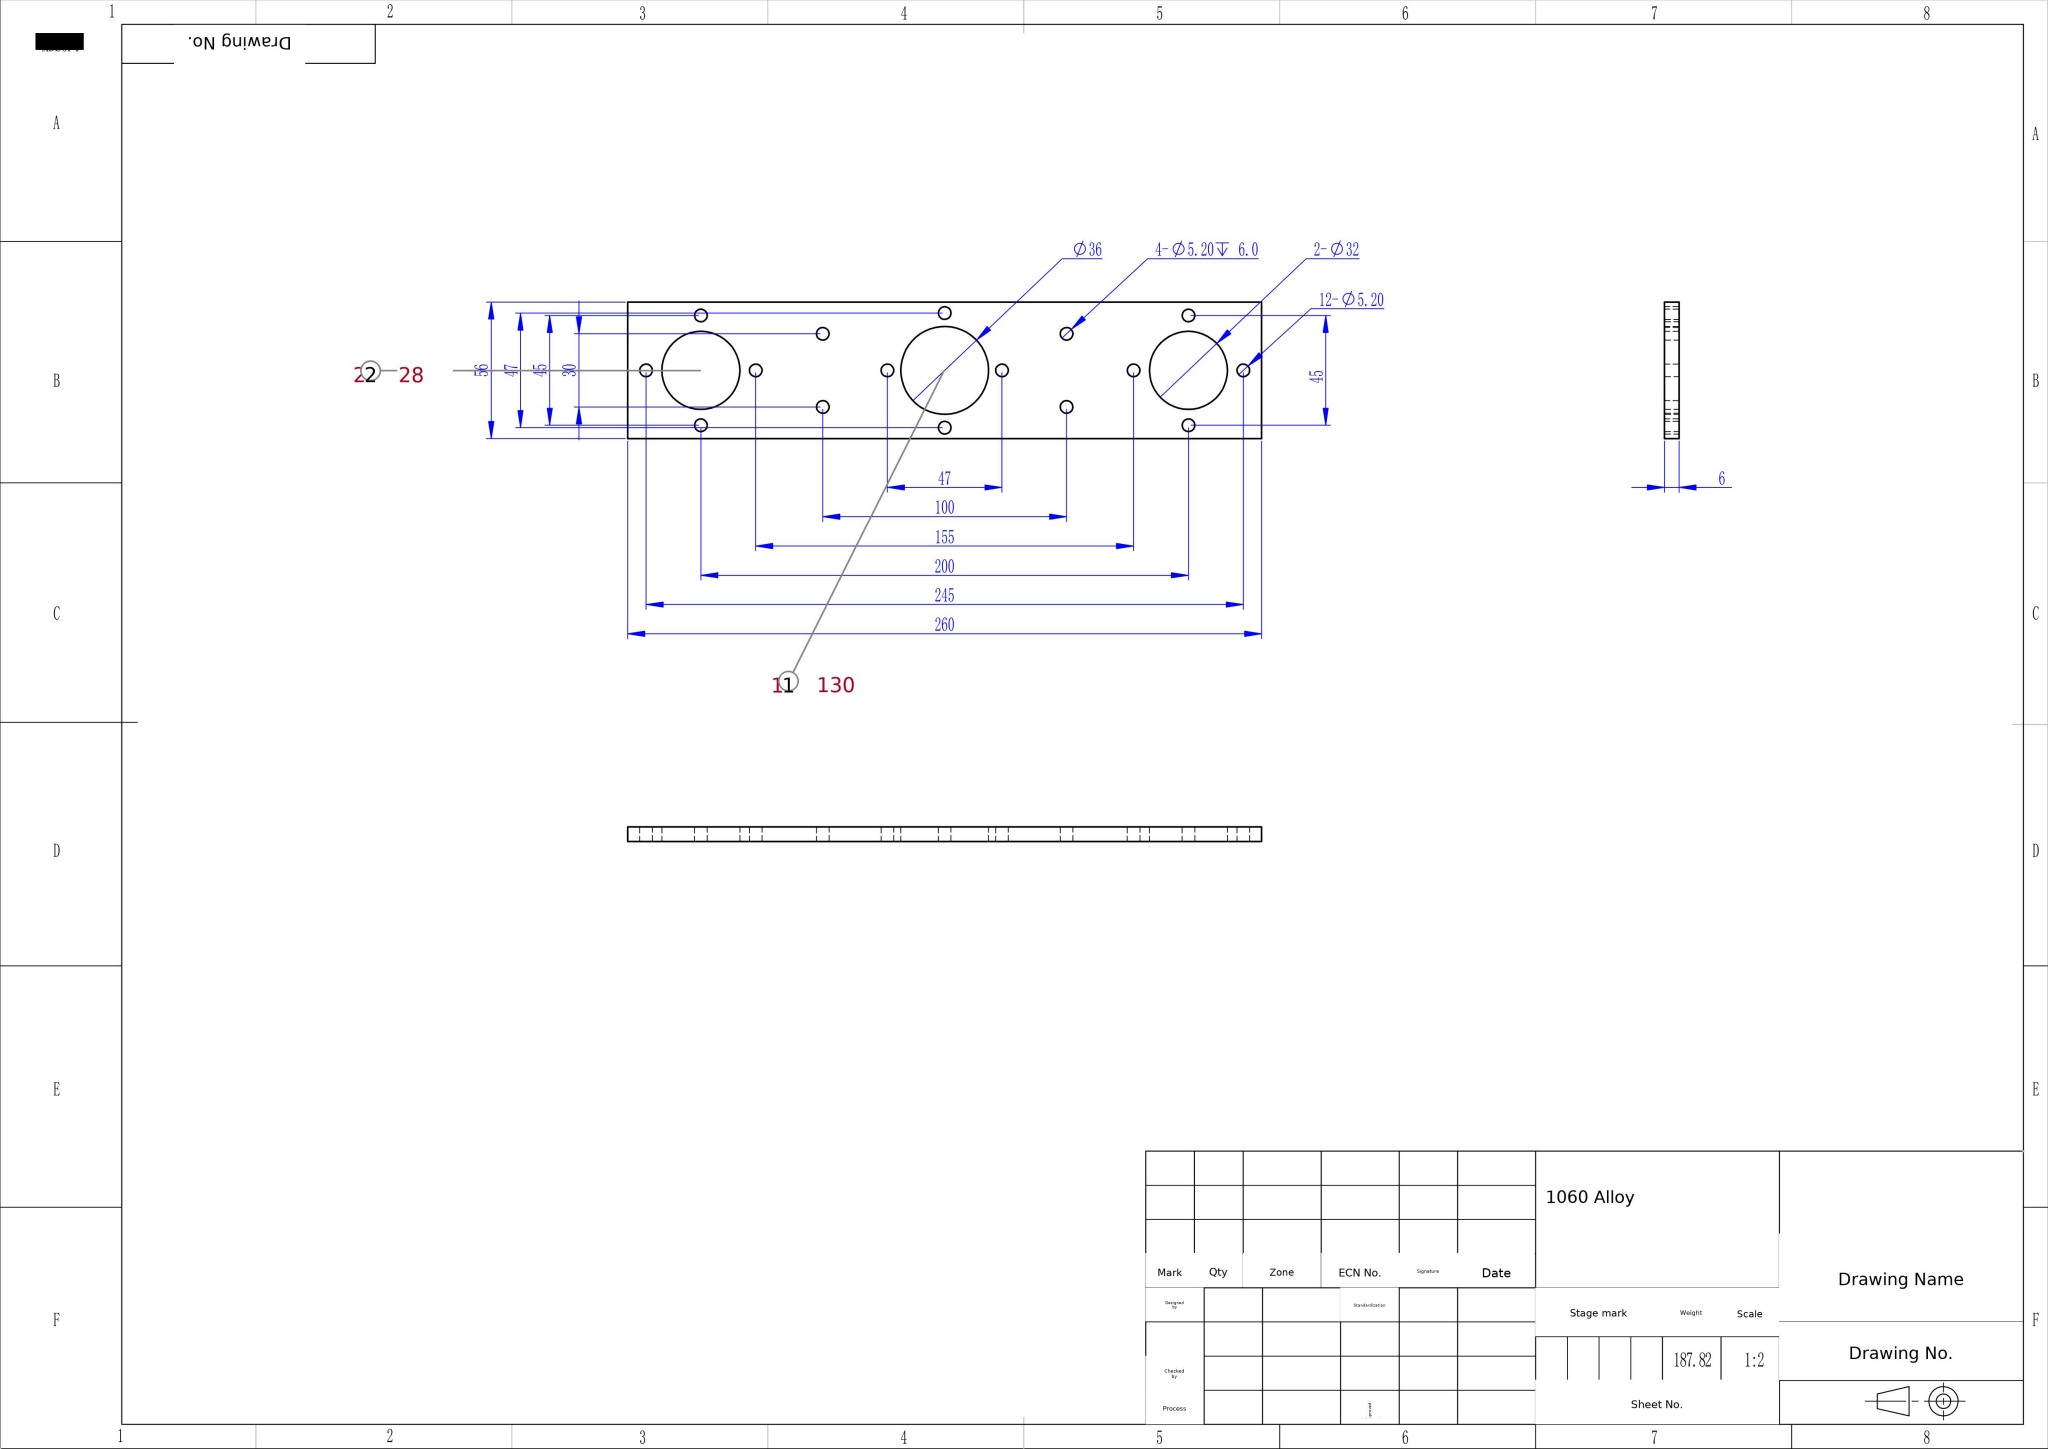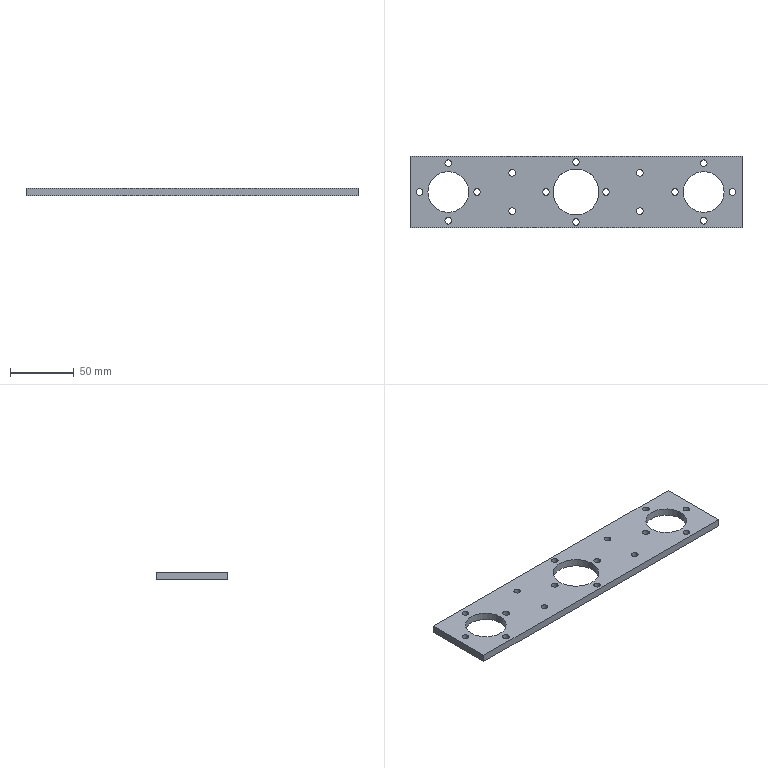Part | SolidWorks | mm | material 1060 Alloy | 1 solid | 44 faces | box 260 x 56 x 6 mm | volume 69563 mm3 | cylinder 38 | plane 6 | commonest cylinder face diameters 5.2 x32 32 x4 36 x2
build123d program:
from build123d import *

# Parameters (mm, degrees)
SKETCH2_W           = 260
SKETCH2_H           = 56
SKETCH2_R           = 18
SKETCH2_R_2         = 2.6
SKETCH2_R_3         = 16
BOSS_EXTRUDE1_DEPTH = 6
SKETCH3_R           = 2.6
CUT_EXTRUDE1_DEPTH  = 6


with BuildPart() as part:
    # Sketch2 → Boss-Extrude1 (new body)
    with BuildSketch(Plane.XY):
        Rectangle(SKETCH2_W, SKETCH2_H)
        Circle(SKETCH2_R, mode=Mode.SUBTRACT)
        with Locations((0, 23.5)):
            Circle(SKETCH2_R_2, mode=Mode.SUBTRACT)
        with Locations((23.5, 0)):
            Circle(SKETCH2_R_2, mode=Mode.SUBTRACT)
        with Locations((0, -23.5)):
            Circle(SKETCH2_R_2, mode=Mode.SUBTRACT)
        with Locations((-23.5, 0)):
            Circle(SKETCH2_R_2, mode=Mode.SUBTRACT)
        with Locations((100, 0)):
            Circle(SKETCH2_R_3, mode=Mode.SUBTRACT)
        with Locations((122.5, 0)):
            Circle(SKETCH2_R_2, mode=Mode.SUBTRACT)
        with Locations((100, -22.5)):
            Circle(SKETCH2_R_2, mode=Mode.SUBTRACT)
        with Locations((77.5, 0)):
            Circle(SKETCH2_R_2, mode=Mode.SUBTRACT)
        with Locations((100, 22.5)):
            Circle(SKETCH2_R_2, mode=Mode.SUBTRACT)
        with Locations(Location((-77.5, 0, 0), (0, 0, 180))):
            Circle(SKETCH2_R_2, mode=Mode.SUBTRACT)
        with Locations(Location((-100, -22.5, 0), (0, 0, 180))):
            Circle(SKETCH2_R_2, mode=Mode.SUBTRACT)
        with Locations(Location((-122.5, 0, 0), (0, 0, 180))):
            Circle(SKETCH2_R_2, mode=Mode.SUBTRACT)
        with Locations(Location((-100, 22.5, 0), (0, 0, 180))):
            Circle(SKETCH2_R_2, mode=Mode.SUBTRACT)
        with Locations(Location((-100, 0, 0), (0, 0, 180))):
            Circle(SKETCH2_R_3, mode=Mode.SUBTRACT)
    extrude(amount=BOSS_EXTRUDE1_DEPTH)

    # Sketch3 → Cut-Extrude1 (cut)
    with BuildSketch(Plane.XY.offset(6)):
        with Locations((-50, 15)):
            Circle(SKETCH3_R)
        with Locations(Location((-50, -15, 0), (0, 0, 180))):
            Circle(SKETCH3_R)
        with Locations((50, -15)):
            Circle(SKETCH3_R)
        with Locations(Location((50, 15, 0), (0, 0, 180))):
            Circle(SKETCH3_R)
    extrude(amount=-CUT_EXTRUDE1_DEPTH, mode=Mode.SUBTRACT)


solid = part.part